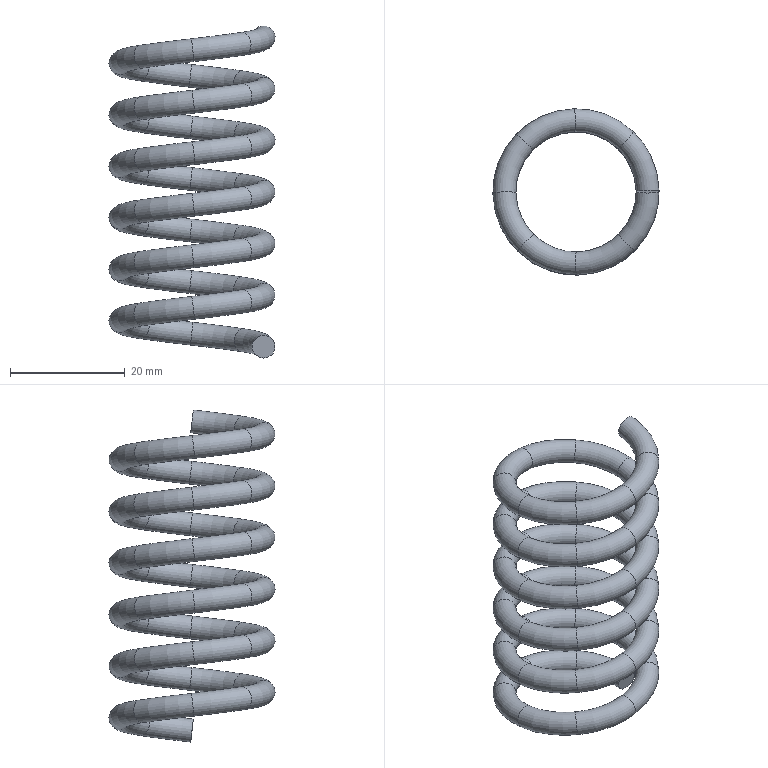Component | NX | SPRING | 1 solid | 50 faces | volume 5960 mm3 | torus 48 | plane 2